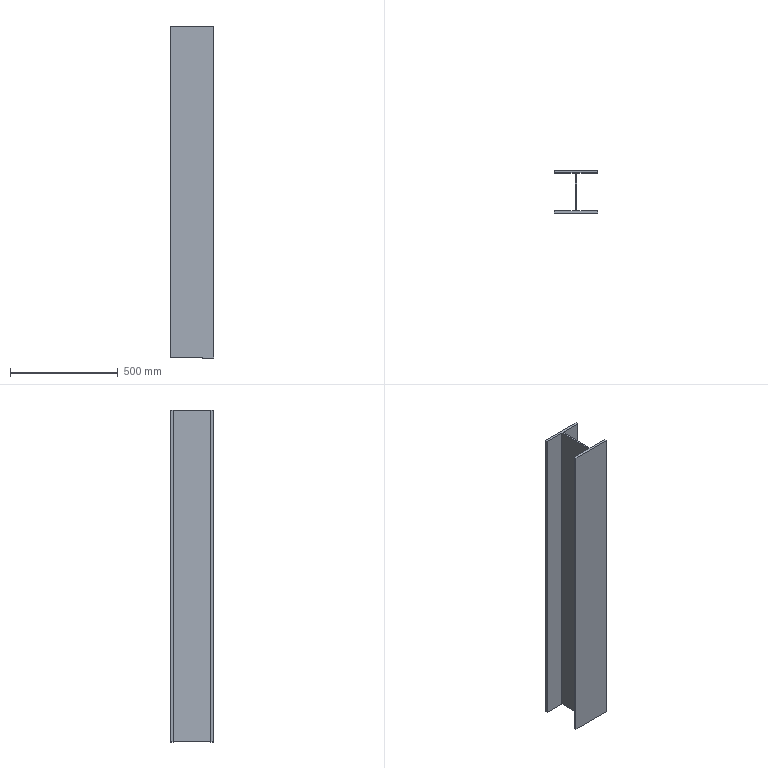Component | SolidWorks | I-Beam200-3 | 1 solid | 14 faces | box 200 x 200 x 1540 mm | volume 9560320 mm3 | plane 14 | material Plain Carbon Steel
build123d program:
from build123d import *

# Parameters (mm, degrees)
BOSS_EXTRUDE1_DEPTH = 1540


with BuildPart() as part:
    # Sketch1 → Boss-Extrude1 (new body)
    with BuildSketch(Plane(origin=(0, 0, 0), x_dir=(1, 0, 0), z_dir=(0, 1, 0))):
        Polygon((0, 0), (0, 200), (12, 200), (12, 104), (188, 104), (188, 200), (200, 200), (200, 0), (188, 0), (188, 96), (12, 96), (12, 0), align=None)
    extrude(amount=BOSS_EXTRUDE1_DEPTH)


solid = part.part

# Placed as in the assembly
solid = solid.moved(Location((16844.937, 3209.803, 2030.287), (90, -90, 0)))
STEP:
#1=COLOUR_RGB('',0.7922,0.8196,0.9333);
#2=FILL_AREA_STYLE_COLOUR('',#1);
#3=FILL_AREA_STYLE('',(#2));
#4=SURFACE_STYLE_FILL_AREA(#3);
#5=SURFACE_SIDE_STYLE('',(#4));
#6=SURFACE_STYLE_USAGE(.BOTH.,#5);
#7=PRESENTATION_STYLE_ASSIGNMENT((#6));
#8=CARTESIAN_POINT('',(671.061,118.496,79.933));
#9=VERTEX_POINT('',#8);
#10=CARTESIAN_POINT('',(671.061,118.969,79.933));
#11=VERTEX_POINT('',#10);
#12=CARTESIAN_POINT('',(671.061,118.969,79.933));
#13=DIRECTION('',(0.,1.,-0.));
#14=VECTOR('',#13,39.37);
#15=LINE('',#12,#14);
#16=EDGE_CURVE('',#9,#11,#15,.T.);
#17=ORIENTED_EDGE('',*,*,#16,.T.);
#18=CARTESIAN_POINT('',(671.061,118.969,140.562));
#19=VERTEX_POINT('',#18);
#20=CARTESIAN_POINT('',(671.061,118.969,140.562));
#21=DIRECTION('',(-0.,-0.,-1.));
#22=VECTOR('',#21,39.37);
#23=LINE('',#20,#22);
#24=EDGE_CURVE('',#19,#11,#23,.T.);
#25=ORIENTED_EDGE('',*,*,#24,.F.);
#26=CARTESIAN_POINT('',(671.061,118.496,140.562));
#27=VERTEX_POINT('',#26);
#28=CARTESIAN_POINT('',(671.061,118.969,140.562));
#29=DIRECTION('',(0.,1.,-0.));
#30=VECTOR('',#29,39.37);
#31=LINE('',#28,#30);
#32=EDGE_CURVE('',#27,#19,#31,.T.);
#33=ORIENTED_EDGE('',*,*,#32,.F.);
#34=CARTESIAN_POINT('',(671.061,118.496,140.562));
#35=DIRECTION('',(-0.,-0.,-1.));
#36=VECTOR('',#35,39.37);
#37=LINE('',#34,#36);
#38=EDGE_CURVE('',#27,#9,#37,.T.);
#39=ORIENTED_EDGE('',*,*,#38,.T.);
#40=EDGE_LOOP('',(#17,#25,#33,#39));
#41=FACE_OUTER_BOUND('',#40,.T.);
#42=CARTESIAN_POINT('',(671.061,118.969,140.562));
#43=DIRECTION('',(-1.,0.,0.));
#44=DIRECTION('',(-0.,-1.,0.));
#45=AXIS2_PLACEMENT_3D('',#42,#43,#44);
#46=PLANE('',#45);
#47=ADVANCED_FACE('',(#41),#46,.F.);
#48=CARTESIAN_POINT('',(667.281,118.969,79.933));
#49=VERTEX_POINT('',#48);
#50=CARTESIAN_POINT('',(667.281,118.969,79.933));
#51=DIRECTION('',(-1.,0.,0.));
#52=VECTOR('',#51,39.37);
#53=LINE('',#50,#52);
#54=EDGE_CURVE('',#11,#49,#53,.T.);
#55=ORIENTED_EDGE('',*,*,#54,.T.);
#56=CARTESIAN_POINT('',(667.281,118.969,140.562));
#57=VERTEX_POINT('',#56);
#58=CARTESIAN_POINT('',(667.281,118.969,140.562));
#59=DIRECTION('',(-0.,-0.,-1.));
#60=VECTOR('',#59,39.37);
#61=LINE('',#58,#60);
#62=EDGE_CURVE('',#57,#49,#61,.T.);
#63=ORIENTED_EDGE('',*,*,#62,.F.);
#64=CARTESIAN_POINT('',(667.281,118.969,140.562));
#65=DIRECTION('',(-1.,0.,0.));
#66=VECTOR('',#65,39.37);
#67=LINE('',#64,#66);
#68=EDGE_CURVE('',#19,#57,#67,.T.);
#69=ORIENTED_EDGE('',*,*,#68,.F.);
#70=ORIENTED_EDGE('',*,*,#24,.T.);
#71=EDGE_LOOP('',(#55,#63,#69,#70));
#72=FACE_OUTER_BOUND('',#71,.T.);
#73=CARTESIAN_POINT('',(667.281,118.969,140.562));
#74=DIRECTION('',(-0.,-1.,0.));
#75=DIRECTION('',(1.,-0.,-0.));
#76=AXIS2_PLACEMENT_3D('',#73,#74,#75);
#77=PLANE('',#76);
#78=ADVANCED_FACE('',(#72),#77,.F.);
#79=CARTESIAN_POINT('',(667.281,125.898,79.933));
#80=VERTEX_POINT('',#79);
#81=CARTESIAN_POINT('',(667.281,125.898,79.933));
#82=DIRECTION('',(0.,1.,-0.));
#83=VECTOR('',#82,39.37);
#84=LINE('',#81,#83);
#85=EDGE_CURVE('',#49,#80,#84,.T.);
#86=ORIENTED_EDGE('',*,*,#85,.T.);
#87=CARTESIAN_POINT('',(667.281,125.898,140.562));
#88=VERTEX_POINT('',#87);
#89=CARTESIAN_POINT('',(667.281,125.898,140.562));
#90=DIRECTION('',(-0.,-0.,-1.));
#91=VECTOR('',#90,39.37);
#92=LINE('',#89,#91);
#93=EDGE_CURVE('',#88,#80,#92,.T.);
#94=ORIENTED_EDGE('',*,*,#93,.F.);
#95=CARTESIAN_POINT('',(667.281,125.898,140.562));
#96=DIRECTION('',(0.,1.,-0.));
#97=VECTOR('',#96,39.37);
#98=LINE('',#95,#97);
#99=EDGE_CURVE('',#57,#88,#98,.T.);
#100=ORIENTED_EDGE('',*,*,#99,.F.);
#101=ORIENTED_EDGE('',*,*,#62,.T.);
#102=EDGE_LOOP('',(#86,#94,#100,#101));
#103=FACE_OUTER_BOUND('',#102,.T.);
#104=CARTESIAN_POINT('',(667.281,125.898,140.562));
#105=DIRECTION('',(-1.,0.,0.));
#106=DIRECTION('',(-0.,-1.,0.));
#107=AXIS2_PLACEMENT_3D('',#104,#105,#106);
#108=PLANE('',#107);
#109=ADVANCED_FACE('',(#103),#108,.F.);
#110=CARTESIAN_POINT('',(671.061,125.898,79.933));
#111=VERTEX_POINT('',#110);
#112=CARTESIAN_POINT('',(671.061,125.898,79.933));
#113=DIRECTION('',(1.,-0.,-0.));
#114=VECTOR('',#113,39.37);
#115=LINE('',#112,#114);
#116=EDGE_CURVE('',#80,#111,#115,.T.);
#117=ORIENTED_EDGE('',*,*,#116,.T.);
#118=CARTESIAN_POINT('',(671.061,125.898,140.562));
#119=VERTEX_POINT('',#118);
#120=CARTESIAN_POINT('',(671.061,125.898,140.562));
#121=DIRECTION('',(-0.,-0.,-1.));
#122=VECTOR('',#121,39.37);
#123=LINE('',#120,#122);
#124=EDGE_CURVE('',#119,#111,#123,.T.);
#125=ORIENTED_EDGE('',*,*,#124,.F.);
#126=CARTESIAN_POINT('',(671.061,125.898,140.562));
#127=DIRECTION('',(1.,-0.,-0.));
#128=VECTOR('',#127,39.37);
#129=LINE('',#126,#128);
#130=EDGE_CURVE('',#88,#119,#129,.T.);
#131=ORIENTED_EDGE('',*,*,#130,.F.);
#132=ORIENTED_EDGE('',*,*,#93,.T.);
#133=EDGE_LOOP('',(#117,#125,#131,#132));
#134=FACE_OUTER_BOUND('',#133,.T.);
#135=CARTESIAN_POINT('',(671.061,125.898,140.562));
#136=DIRECTION('',(0.,1.,-0.));
#137=DIRECTION('',(-1.,0.,0.));
#138=AXIS2_PLACEMENT_3D('',#135,#136,#137);
#139=PLANE('',#138);
#140=ADVANCED_FACE('',(#134),#139,.F.);
#141=CARTESIAN_POINT('',(671.061,126.37,79.933));
#142=VERTEX_POINT('',#141);
#143=CARTESIAN_POINT('',(671.061,126.37,79.933));
#144=DIRECTION('',(0.,1.,-0.));
#145=VECTOR('',#144,39.37);
#146=LINE('',#143,#145);
#147=EDGE_CURVE('',#111,#142,#146,.T.);
#148=ORIENTED_EDGE('',*,*,#147,.T.);
#149=CARTESIAN_POINT('',(671.061,126.37,140.562));
#150=VERTEX_POINT('',#149);
#151=CARTESIAN_POINT('',(671.061,126.37,140.562));
#152=DIRECTION('',(-0.,-0.,-1.));
#153=VECTOR('',#152,39.37);
#154=LINE('',#151,#153);
#155=EDGE_CURVE('',#150,#142,#154,.T.);
#156=ORIENTED_EDGE('',*,*,#155,.F.);
#157=CARTESIAN_POINT('',(671.061,126.37,140.562));
#158=DIRECTION('',(0.,1.,-0.));
#159=VECTOR('',#158,39.37);
#160=LINE('',#157,#159);
#161=EDGE_CURVE('',#119,#150,#160,.T.);
#162=ORIENTED_EDGE('',*,*,#161,.F.);
#163=ORIENTED_EDGE('',*,*,#124,.T.);
#164=EDGE_LOOP('',(#148,#156,#162,#163));
#165=FACE_OUTER_BOUND('',#164,.T.);
#166=CARTESIAN_POINT('',(671.061,126.37,140.562));
#167=DIRECTION('',(-1.,0.,0.));
#168=DIRECTION('',(-0.,-1.,0.));
#169=AXIS2_PLACEMENT_3D('',#166,#167,#168);
#170=PLANE('',#169);
#171=ADVANCED_FACE('',(#165),#170,.F.);
#172=CARTESIAN_POINT('',(663.187,126.37,79.933));
#173=VERTEX_POINT('',#172);
#174=CARTESIAN_POINT('',(663.187,126.37,79.933));
#175=DIRECTION('',(-1.,0.,0.));
#176=VECTOR('',#175,39.37);
#177=LINE('',#174,#176);
#178=EDGE_CURVE('',#142,#173,#177,.T.);
#179=ORIENTED_EDGE('',*,*,#178,.T.);
#180=CARTESIAN_POINT('',(663.187,126.37,140.562));
#181=VERTEX_POINT('',#180);
#182=CARTESIAN_POINT('',(663.187,126.37,140.562));
#183=DIRECTION('',(-0.,-0.,-1.));
#184=VECTOR('',#183,39.37);
#185=LINE('',#182,#184);
#186=EDGE_CURVE('',#181,#173,#185,.T.);
#187=ORIENTED_EDGE('',*,*,#186,.F.);
#188=CARTESIAN_POINT('',(663.187,126.37,140.562));
#189=DIRECTION('',(-1.,0.,0.));
#190=VECTOR('',#189,39.37);
#191=LINE('',#188,#190);
#192=EDGE_CURVE('',#150,#181,#191,.T.);
#193=ORIENTED_EDGE('',*,*,#192,.F.);
#194=ORIENTED_EDGE('',*,*,#155,.T.);
#195=EDGE_LOOP('',(#179,#187,#193,#194));
#196=FACE_OUTER_BOUND('',#195,.T.);
#197=CARTESIAN_POINT('',(663.187,126.37,140.562));
#198=DIRECTION('',(-0.,-1.,0.));
#199=DIRECTION('',(1.,-0.,-0.));
#200=AXIS2_PLACEMENT_3D('',#197,#198,#199);
#201=PLANE('',#200);
#202=ADVANCED_FACE('',(#196),#201,.F.);
#203=CARTESIAN_POINT('',(663.187,125.898,79.933));
#204=VERTEX_POINT('',#203);
#205=CARTESIAN_POINT('',(663.187,125.898,79.933));
#206=DIRECTION('',(-0.,-1.,0.));
#207=VECTOR('',#206,39.37);
#208=LINE('',#205,#207);
#209=EDGE_CURVE('',#173,#204,#208,.T.);
#210=ORIENTED_EDGE('',*,*,#209,.T.);
#211=CARTESIAN_POINT('',(663.187,125.898,140.562));
#212=VERTEX_POINT('',#211);
#213=CARTESIAN_POINT('',(663.187,125.898,140.562));
#214=DIRECTION('',(-0.,-0.,-1.));
#215=VECTOR('',#214,39.37);
#216=LINE('',#213,#215);
#217=EDGE_CURVE('',#212,#204,#216,.T.);
#218=ORIENTED_EDGE('',*,*,#217,.F.);
#219=CARTESIAN_POINT('',(663.187,125.898,140.562));
#220=DIRECTION('',(-0.,-1.,0.));
#221=VECTOR('',#220,39.37);
#222=LINE('',#219,#221);
#223=EDGE_CURVE('',#181,#212,#222,.T.);
#224=ORIENTED_EDGE('',*,*,#223,.F.);
#225=ORIENTED_EDGE('',*,*,#186,.T.);
#226=EDGE_LOOP('',(#210,#218,#224,#225));
#227=FACE_OUTER_BOUND('',#226,.T.);
#228=CARTESIAN_POINT('',(663.187,125.898,140.562));
#229=DIRECTION('',(1.,-0.,-0.));
#230=DIRECTION('',(0.,1.,-0.));
#231=AXIS2_PLACEMENT_3D('',#228,#229,#230);
#232=PLANE('',#231);
#233=ADVANCED_FACE('',(#227),#232,.F.);
#234=CARTESIAN_POINT('',(666.966,125.898,79.933));
#235=VERTEX_POINT('',#234);
#236=CARTESIAN_POINT('',(666.966,125.898,79.933));
#237=DIRECTION('',(1.,-0.,-0.));
#238=VECTOR('',#237,39.37);
#239=LINE('',#236,#238);
#240=EDGE_CURVE('',#204,#235,#239,.T.);
#241=ORIENTED_EDGE('',*,*,#240,.T.);
#242=CARTESIAN_POINT('',(666.966,125.898,140.562));
#243=VERTEX_POINT('',#242);
#244=CARTESIAN_POINT('',(666.966,125.898,140.562));
#245=DIRECTION('',(-0.,-0.,-1.));
#246=VECTOR('',#245,39.37);
#247=LINE('',#244,#246);
#248=EDGE_CURVE('',#243,#235,#247,.T.);
#249=ORIENTED_EDGE('',*,*,#248,.F.);
#250=CARTESIAN_POINT('',(666.966,125.898,140.562));
#251=DIRECTION('',(1.,-0.,-0.));
#252=VECTOR('',#251,39.37);
#253=LINE('',#250,#252);
#254=EDGE_CURVE('',#212,#243,#253,.T.);
#255=ORIENTED_EDGE('',*,*,#254,.F.);
#256=ORIENTED_EDGE('',*,*,#217,.T.);
#257=EDGE_LOOP('',(#241,#249,#255,#256));
#258=FACE_OUTER_BOUND('',#257,.T.);
#259=CARTESIAN_POINT('',(666.966,125.898,140.562));
#260=DIRECTION('',(0.,1.,-0.));
#261=DIRECTION('',(-1.,0.,0.));
#262=AXIS2_PLACEMENT_3D('',#259,#260,#261);
#263=PLANE('',#262);
#264=ADVANCED_FACE('',(#258),#263,.F.);
#265=CARTESIAN_POINT('',(666.966,118.969,79.933));
#266=VERTEX_POINT('',#265);
#267=CARTESIAN_POINT('',(666.966,118.969,79.933));
#268=DIRECTION('',(-0.,-1.,0.));
#269=VECTOR('',#268,39.37);
#270=LINE('',#267,#269);
#271=EDGE_CURVE('',#235,#266,#270,.T.);
#272=ORIENTED_EDGE('',*,*,#271,.T.);
#273=CARTESIAN_POINT('',(666.966,118.969,140.562));
#274=VERTEX_POINT('',#273);
#275=CARTESIAN_POINT('',(666.966,118.969,140.562));
#276=DIRECTION('',(-0.,-0.,-1.));
#277=VECTOR('',#276,39.37);
#278=LINE('',#275,#277);
#279=EDGE_CURVE('',#274,#266,#278,.T.);
#280=ORIENTED_EDGE('',*,*,#279,.F.);
#281=CARTESIAN_POINT('',(666.966,118.969,140.562));
#282=DIRECTION('',(-0.,-1.,0.));
#283=VECTOR('',#282,39.37);
#284=LINE('',#281,#283);
#285=EDGE_CURVE('',#243,#274,#284,.T.);
#286=ORIENTED_EDGE('',*,*,#285,.F.);
#287=ORIENTED_EDGE('',*,*,#248,.T.);
#288=EDGE_LOOP('',(#272,#280,#286,#287));
#289=FACE_OUTER_BOUND('',#288,.T.);
#290=CARTESIAN_POINT('',(666.966,118.969,140.562));
#291=DIRECTION('',(1.,-0.,-0.));
#292=DIRECTION('',(0.,1.,-0.));
#293=AXIS2_PLACEMENT_3D('',#290,#291,#292);
#294=PLANE('',#293);
#295=ADVANCED_FACE('',(#289),#294,.F.);
#296=CARTESIAN_POINT('',(663.187,118.969,79.933));
#297=VERTEX_POINT('',#296);
#298=CARTESIAN_POINT('',(663.187,118.969,79.933));
#299=DIRECTION('',(-1.,0.,0.));
#300=VECTOR('',#299,39.37);
#301=LINE('',#298,#300);
#302=EDGE_CURVE('',#266,#297,#301,.T.);
#303=ORIENTED_EDGE('',*,*,#302,.T.);
#304=CARTESIAN_POINT('',(663.187,118.969,140.562));
#305=VERTEX_POINT('',#304);
#306=CARTESIAN_POINT('',(663.187,118.969,140.562));
#307=DIRECTION('',(-0.,-0.,-1.));
#308=VECTOR('',#307,39.37);
#309=LINE('',#306,#308);
#310=EDGE_CURVE('',#305,#297,#309,.T.);
#311=ORIENTED_EDGE('',*,*,#310,.F.);
#312=CARTESIAN_POINT('',(663.187,118.969,140.562));
#313=DIRECTION('',(-1.,0.,0.));
#314=VECTOR('',#313,39.37);
#315=LINE('',#312,#314);
#316=EDGE_CURVE('',#274,#305,#315,.T.);
#317=ORIENTED_EDGE('',*,*,#316,.F.);
#318=ORIENTED_EDGE('',*,*,#279,.T.);
#319=EDGE_LOOP('',(#303,#311,#317,#318));
#320=FACE_OUTER_BOUND('',#319,.T.);
#321=CARTESIAN_POINT('',(663.187,118.969,140.562));
#322=DIRECTION('',(-0.,-1.,0.));
#323=DIRECTION('',(1.,-0.,-0.));
#324=AXIS2_PLACEMENT_3D('',#321,#322,#323);
#325=PLANE('',#324);
#326=ADVANCED_FACE('',(#320),#325,.F.);
#327=CARTESIAN_POINT('',(663.187,118.496,79.933));
#328=VERTEX_POINT('',#327);
#329=CARTESIAN_POINT('',(663.187,118.496,79.933));
#330=DIRECTION('',(-0.,-1.,0.));
#331=VECTOR('',#330,39.37);
#332=LINE('',#329,#331);
#333=EDGE_CURVE('',#297,#328,#332,.T.);
#334=ORIENTED_EDGE('',*,*,#333,.T.);
#335=CARTESIAN_POINT('',(663.187,118.496,140.562));
#336=VERTEX_POINT('',#335);
#337=CARTESIAN_POINT('',(663.187,118.496,140.562));
#338=DIRECTION('',(-0.,-0.,-1.));
#339=VECTOR('',#338,39.37);
#340=LINE('',#337,#339);
#341=EDGE_CURVE('',#336,#328,#340,.T.);
#342=ORIENTED_EDGE('',*,*,#341,.F.);
#343=CARTESIAN_POINT('',(663.187,118.496,140.562));
#344=DIRECTION('',(-0.,-1.,0.));
#345=VECTOR('',#344,39.37);
#346=LINE('',#343,#345);
#347=EDGE_CURVE('',#305,#336,#346,.T.);
#348=ORIENTED_EDGE('',*,*,#347,.F.);
#349=ORIENTED_EDGE('',*,*,#310,.T.);
#350=EDGE_LOOP('',(#334,#342,#348,#349));
#351=FACE_OUTER_BOUND('',#350,.T.);
#352=CARTESIAN_POINT('',(663.187,118.496,140.562));
#353=DIRECTION('',(1.,-0.,-0.));
#354=DIRECTION('',(0.,1.,-0.));
#355=AXIS2_PLACEMENT_3D('',#352,#353,#354);
#356=PLANE('',#355);
#357=ADVANCED_FACE('',(#351),#356,.F.);
#358=CARTESIAN_POINT('',(671.061,118.496,79.933));
#359=DIRECTION('',(1.,-0.,-0.));
#360=VECTOR('',#359,39.37);
#361=LINE('',#358,#360);
#362=EDGE_CURVE('',#328,#9,#361,.T.);
#363=ORIENTED_EDGE('',*,*,#362,.T.);
#364=ORIENTED_EDGE('',*,*,#38,.F.);
#365=CARTESIAN_POINT('',(671.061,118.496,140.562));
#366=DIRECTION('',(1.,-0.,-0.));
#367=VECTOR('',#366,39.37);
#368=LINE('',#365,#367);
#369=EDGE_CURVE('',#336,#27,#368,.T.);
#370=ORIENTED_EDGE('',*,*,#369,.F.);
#371=ORIENTED_EDGE('',*,*,#341,.T.);
#372=EDGE_LOOP('',(#363,#364,#370,#371));
#373=FACE_OUTER_BOUND('',#372,.T.);
#374=CARTESIAN_POINT('',(671.061,118.496,140.562));
#375=DIRECTION('',(0.,1.,-0.));
#376=DIRECTION('',(-1.,0.,0.));
#377=AXIS2_PLACEMENT_3D('',#374,#375,#376);
#378=PLANE('',#377);
#379=ADVANCED_FACE('',(#373),#378,.F.);
#380=ORIENTED_EDGE('',*,*,#32,.T.);
#381=ORIENTED_EDGE('',*,*,#68,.T.);
#382=ORIENTED_EDGE('',*,*,#99,.T.);
#383=ORIENTED_EDGE('',*,*,#130,.T.);
#384=ORIENTED_EDGE('',*,*,#161,.T.);
#385=ORIENTED_EDGE('',*,*,#192,.T.);
#386=ORIENTED_EDGE('',*,*,#223,.T.);
#387=ORIENTED_EDGE('',*,*,#254,.T.);
#388=ORIENTED_EDGE('',*,*,#285,.T.);
#389=ORIENTED_EDGE('',*,*,#316,.T.);
#390=ORIENTED_EDGE('',*,*,#347,.T.);
#391=ORIENTED_EDGE('',*,*,#369,.T.);
#392=EDGE_LOOP('',(#380,#381,#382,#383,#384,#385,#386,#387,#388,#389,#390,#391));
#393=FACE_OUTER_BOUND('',#392,.T.);
#394=CARTESIAN_POINT('',(671.061,118.496,140.562));
#395=DIRECTION('',(-0.,-0.,-1.));
#396=DIRECTION('',(-1.,0.,0.));
#397=AXIS2_PLACEMENT_3D('',#394,#395,#396);
#398=PLANE('',#397);
#399=ADVANCED_FACE('',(#393),#398,.F.);
#400=ORIENTED_EDGE('',*,*,#16,.F.);
#401=ORIENTED_EDGE('',*,*,#362,.F.);
#402=ORIENTED_EDGE('',*,*,#333,.F.);
#403=ORIENTED_EDGE('',*,*,#302,.F.);
#404=ORIENTED_EDGE('',*,*,#271,.F.);
#405=ORIENTED_EDGE('',*,*,#240,.F.);
#406=ORIENTED_EDGE('',*,*,#209,.F.);
#407=ORIENTED_EDGE('',*,*,#178,.F.);
#408=ORIENTED_EDGE('',*,*,#147,.F.);
#409=ORIENTED_EDGE('',*,*,#116,.F.);
#410=ORIENTED_EDGE('',*,*,#85,.F.);
#411=ORIENTED_EDGE('',*,*,#54,.F.);
#412=EDGE_LOOP('',(#400,#401,#402,#403,#404,#405,#406,#407,#408,#409,#410,#411));
#413=FACE_OUTER_BOUND('',#412,.T.);
#414=CARTESIAN_POINT('',(671.061,118.496,79.933));
#415=DIRECTION('',(-0.,-0.,-1.));
#416=DIRECTION('',(-1.,0.,0.));
#417=AXIS2_PLACEMENT_3D('',#414,#415,#416);
#418=PLANE('',#417);
#419=ADVANCED_FACE('',(#413),#418,.T.);
#420=CLOSED_SHELL('',(#47,#78,#109,#140,#171,#202,#233,#264,#295,#326,#357,#379,#399,#419));
#421=MANIFOLD_SOLID_BREP('',#420);
#422=STYLED_ITEM('',(#7),#421);
#423=(LENGTH_UNIT()NAMED_UNIT(*)SI_UNIT($,.METRE.));
#424=LENGTH_MEASURE_WITH_UNIT(LENGTH_MEASURE(0.0254),#423);
#425=DIMENSIONAL_EXPONENTS(1.,0.,0.,0.,0.,0.,0.);
#426=(CONVERSION_BASED_UNIT('',#424)LENGTH_UNIT()NAMED_UNIT(#425));
#427=UNCERTAINTY_MEASURE_WITH_UNIT(LENGTH_MEASURE(0.00001),#426,'','');
#428=(NAMED_UNIT(*)PLANE_ANGLE_UNIT()SI_UNIT($,.RADIAN.));
#429=(NAMED_UNIT(*)SI_UNIT($,.STERADIAN.)SOLID_ANGLE_UNIT());
#430=(GEOMETRIC_REPRESENTATION_CONTEXT(3)GLOBAL_UNCERTAINTY_ASSIGNED_CONTEXT((#427))GLOBAL_UNIT_ASSIGNED_CONTEXT((#426,#428,#429))REPRESENTATION_CONTEXT('',''));
#431=MECHANICAL_DESIGN_GEOMETRIC_PRESENTATION_REPRESENTATION('',(#422),#430);
#432=CARTESIAN_POINT('',(0.,0.,0.));
#433=DIRECTION('',(0.,0.,1.));
#434=DIRECTION('',(1.,0.,0.));
#435=AXIS2_PLACEMENT_3D('',#432,#433,#434);
#436=(LENGTH_UNIT()NAMED_UNIT(*)SI_UNIT($,.METRE.));
#437=LENGTH_MEASURE_WITH_UNIT(LENGTH_MEASURE(0.0254),#436);
#438=DIMENSIONAL_EXPONENTS(1.,0.,0.,0.,0.,0.,0.);
#439=(CONVERSION_BASED_UNIT('',#437)LENGTH_UNIT()NAMED_UNIT(#438));
#440=UNCERTAINTY_MEASURE_WITH_UNIT(LENGTH_MEASURE(0.00001),#439,'','');
#441=(NAMED_UNIT(*)PLANE_ANGLE_UNIT()SI_UNIT($,.RADIAN.));
#442=(NAMED_UNIT(*)SI_UNIT($,.STERADIAN.)SOLID_ANGLE_UNIT());
#443=(GEOMETRIC_REPRESENTATION_CONTEXT(3)GLOBAL_UNCERTAINTY_ASSIGNED_CONTEXT((#440))GLOBAL_UNIT_ASSIGNED_CONTEXT((#439,#441,#442))REPRESENTATION_CONTEXT('',''));
#444=ADVANCED_BREP_SHAPE_REPRESENTATION('',(#421,#435),#443);
#445=PRESENTATION_LAYER_ASSIGNMENT('','',(#422));